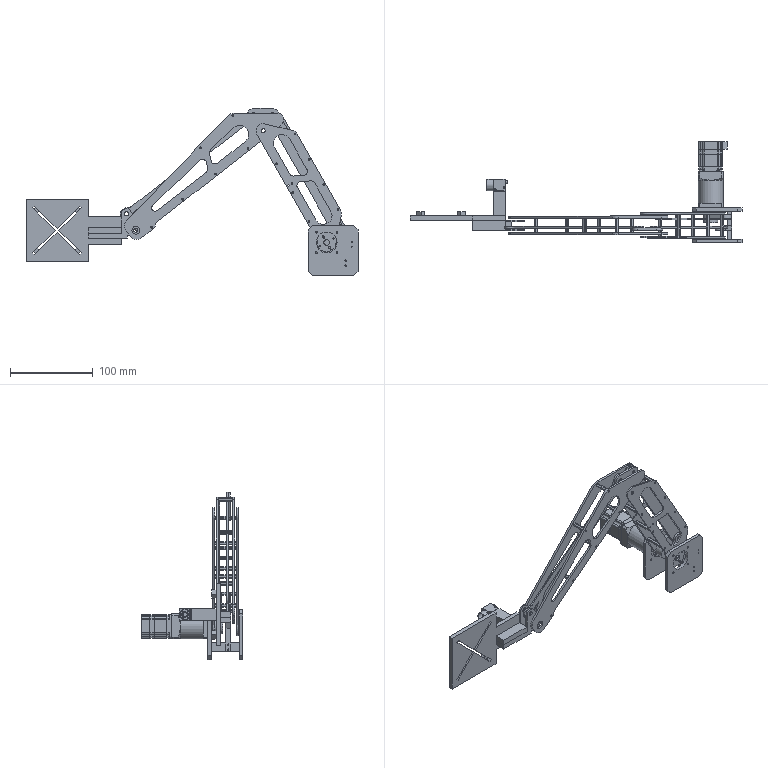Assembly | NX | mm | 31 component files | 44 solids | 1166 faces | box 400.71 x 122.5 x 201.68 mm | volume 207632 mm3 | plane 801 | cylinder 320 | cone 30 | spline 8 | sphere 7 | commonest cylinder face diameters 2.1 x38 3 x37 5 x19 10 x19 1.25 x18 1.65 x17 4.65 x16 2.6 x11
Bill of materials:
unnamed part 1 | 2 |  | Flat, nearly square plate with all four corners chamfered. It has one large circular through-opening offset toward one corner, four small holes in a square pattern around that opening, and two pairs of smaller holes near the opposite edges.
unnamed part 2 | 1 |  | Solid rectangular bar with two holes in one end face and two cross holes through one long side face.
unnamed part 3 | 1 |  | Lever-type link: a flat plate with rounded (obround) ends, with a round boss sticking out from one side at one end. The boss has a through bore, and the plate has a second, smaller hole at the other end.
unnamed part 4 | 1 |  | Clevis-style bracket: a flat rectangular base bar with two parallel triangular lugs standing up at one end. Each lug has two holes, and the base has a pattern of small holes.
unnamed part 5 | 1 |  | Flat triangular plate with rounded corners and three through holes, one near each corner: two smaller holes of equal size and one larger hole.
unnamed part 6 | 2 |  | Thin, long, angled plate with rounded ends and two large rounded-slot cutouts separated by a cross web. It has a larger hole at each end and many small holes along the edges.
unnamed part 7 | 1 |  | Thin, flat Y-shaped strap: a long straight arm and a short branch arm. Each of the three arm ends finishes in a round eye with a hole.
unnamed part 8 | 1 |  | Plate-and-block body: a square flat plate with a rectangular tab sticking out from one side and a thicker rectangular block under the tab region. The plate has X-shaped diagonal slots through it and small diagonal features at the four corners.
unnamed part 9 | 1 |  | Rectangular box-shaped enclosure with a large cylindrical protrusion on one end. A small round connector-like boss with several pin-like features sticks out from a side face. The surfaces show cross-recess screw heads, semicircular notches, round recesses, a rectangular recess and small holes.
unnamed part 10 | 1 |  | Thin, flat, long triangular arm with rounded ends. It has two tapered lightening-style cutouts, a larger hole at each end, and small holes along the edges.
unnamed part 11 | 1 |  | Thin, flat, long triangular arm with rounded ends. It has two tapered lightening-style cutouts, a larger hole at each end, and small holes along the edges, plus one extra small hole at the wide-end corner.
unnamed part 12 | 6 |  | Hexagonal prism with a round bore along its full length.
unnamed part 13 | 7 |  | Long, straight hexagonal bar with a round hole along its central axis. It looks like a hex standoff or spacer.
unnamed part 14 | 2 |  | Thin, flat, straight strip with rounded ends and one round hole near each end. The two holes are different sizes. It looks like a link plate.
unnamed part 15 | 1 |  | Square-flanged body with a single round shaft sticking out of the front face. It looks like a motor. The housing has rounded corners and grooves running along its length. A rectangular block sticks out from one side near the back end.
unnamed part 16 | 1 |  | Housing with square end blocks at both ends and a round body in between. A stepped round shaft sticks out of the front end. It looks like an inline gearbox or reducer.
unnamed part 17 | 1 |  | Flat, bent-profile arm or lever bracket. It has a rounded eye with a large hole at one end, then an angled section, then a straight section. The straight section narrows to a smaller tab with two small cross holes. The thickness is stepped.
Mates:
1. concentric | Motor 1 edge | Motor_Mount 1 edge
2. concentric | 11 1 edge | 1 2 edge
3. concentric | 6 1 edge | 11 1 edge
4. concentric | 8 2 edge | 6 1 edge
5. concentric | 12 7 edge | 2 2 edge
6. concentric | 12 6 edge | 2 2 edge
7. concentric | 12 5 edge | 2 2 edge
8. concentric | 12 4 edge | 2 2 edge
9. concentric | 12 3 edge | 2 2 edge
10. concentric | 12 2 edge | 2 2 edge
11. concentric | 12 1 edge | 2 2 edge
12. concentric | 2 1 edge | 12 7 edge
13. concentric | 2 1 edge | 12 6 edge
14. touch align | 2 1 face | Motor_Mount 1 face
15. concentric | 9 1 edge | 2 1 edge
16. concentric | 13 6 edge | 3 1 edge
17. concentric | 13 1 edge | 3 1 edge
18. concentric | 13 2 edge | 3 1 edge
19. concentric | 13 5 edge | 3 1 edge
20. concentric | 13 4 edge | 3 1 edge
21. concentric | 13 3 edge | 3 1 edge
22. concentric | 8 1 edge | 9 1 edge
23. concentric | mirror_3 1 edge | 13 3 edge
24. concentric | mirror_3 1 edge | 13 6 edge
25. touch align | 3 1 face | 2 2 face
26. concentric | mirror_3 1 edge | 8 1 edge
27. touch align | 4 1 face | 3 1 face
28. touch align | 7 1 face | 2 2 face
29. parallel | 3 1 face | 1 2 face
30. center | 4 1 face | 4 1 face | 3 1 face | mirror_3 1 face
31. touch align | Vision_Camera 1 face | 15 1 face
32. center | Vision_Camera 1 face | Vision_Camera 1 face | 15 1 face | 15 1 face
33. touch align | Vision_Camera 1 face | 15 1 face
34. touch align | 15 1 face | 4 1 face
35. touch align | 15 1 face | 4 1 face
36. concentric | 1 1 edge | 11 1 edge